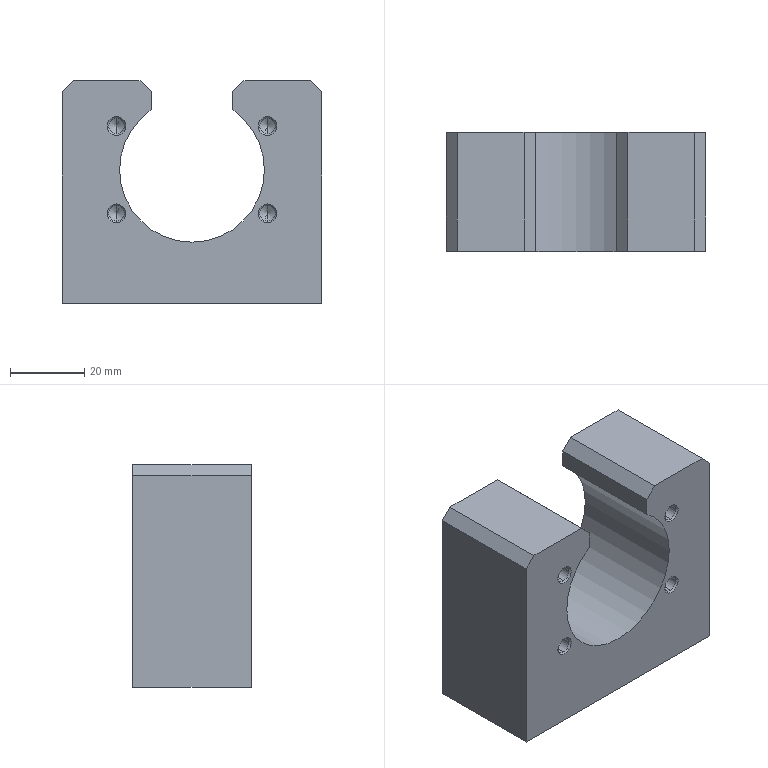CAM job | Mastercam | mm | 9 operations | part box 70 x 32 x 60
1. Facing | 20 - 63 平铣刀
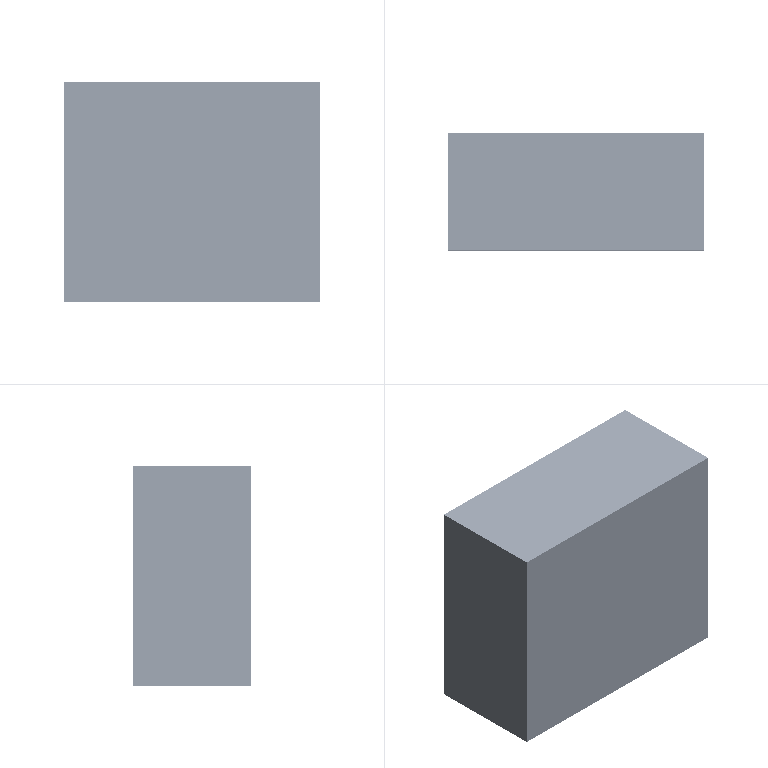2. 2D High Speed (2D Dynamic Mill) | 9 - 10 平铣刀
3. Contour (2D) | 10 - 10 平铣刀
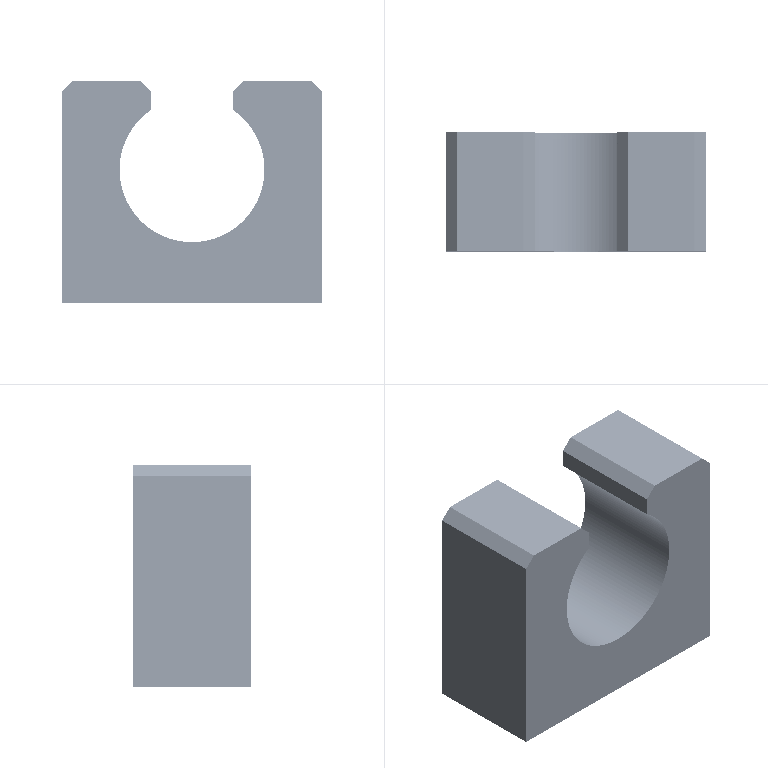4. Contour (Ramp) | 10 - 10 平铣刀
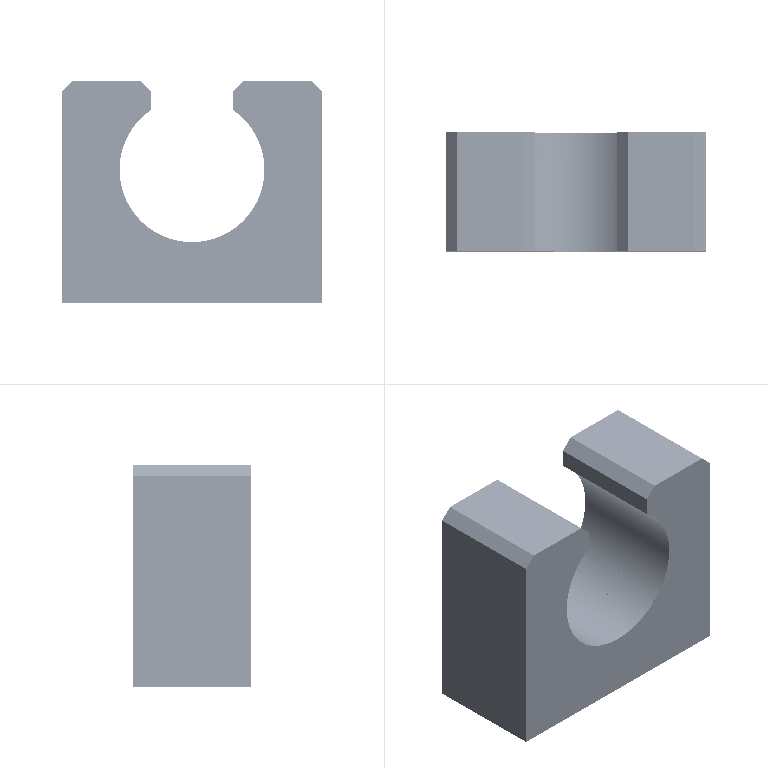5. Contour (2D chamfer) | 7 - 4 倒角刀
6. Facing | 20 - 63 平铣刀
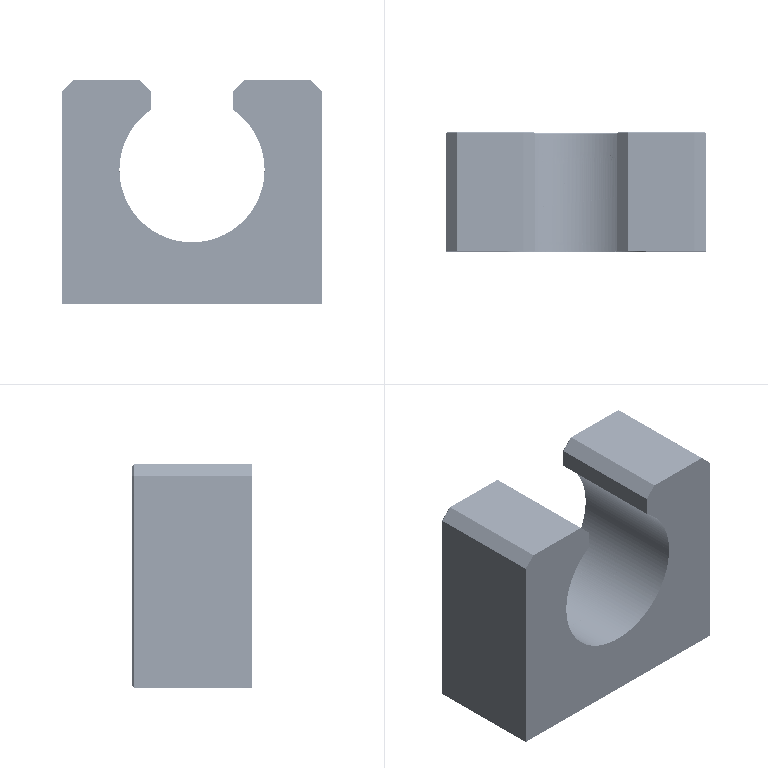7. Contour (2D chamfer) | 7 - 4 倒角刀
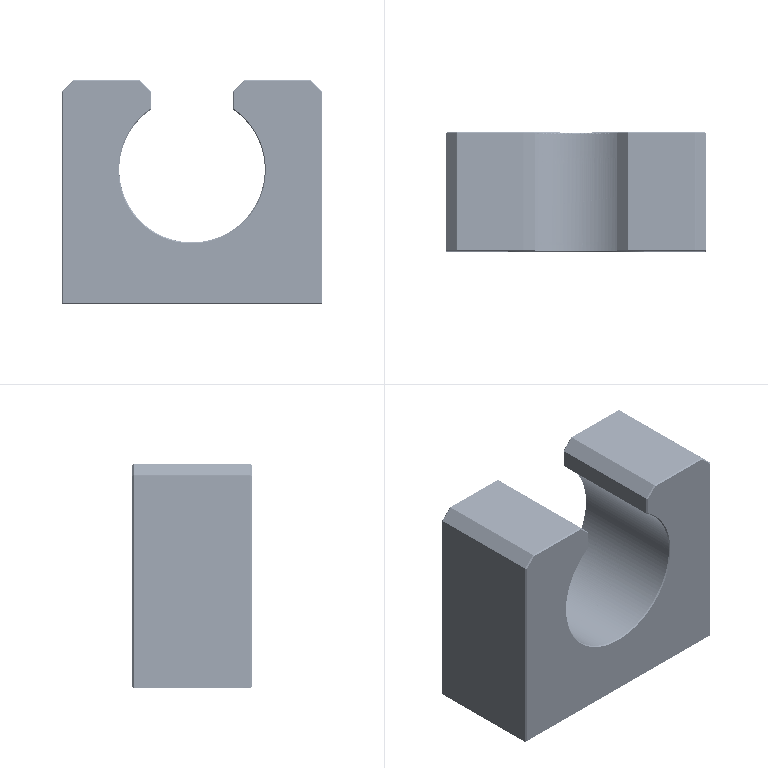8. Drill/Counterbore | 7 - 4 倒角刀
9. Drill/Counterbore | 7 - 4 倒角刀